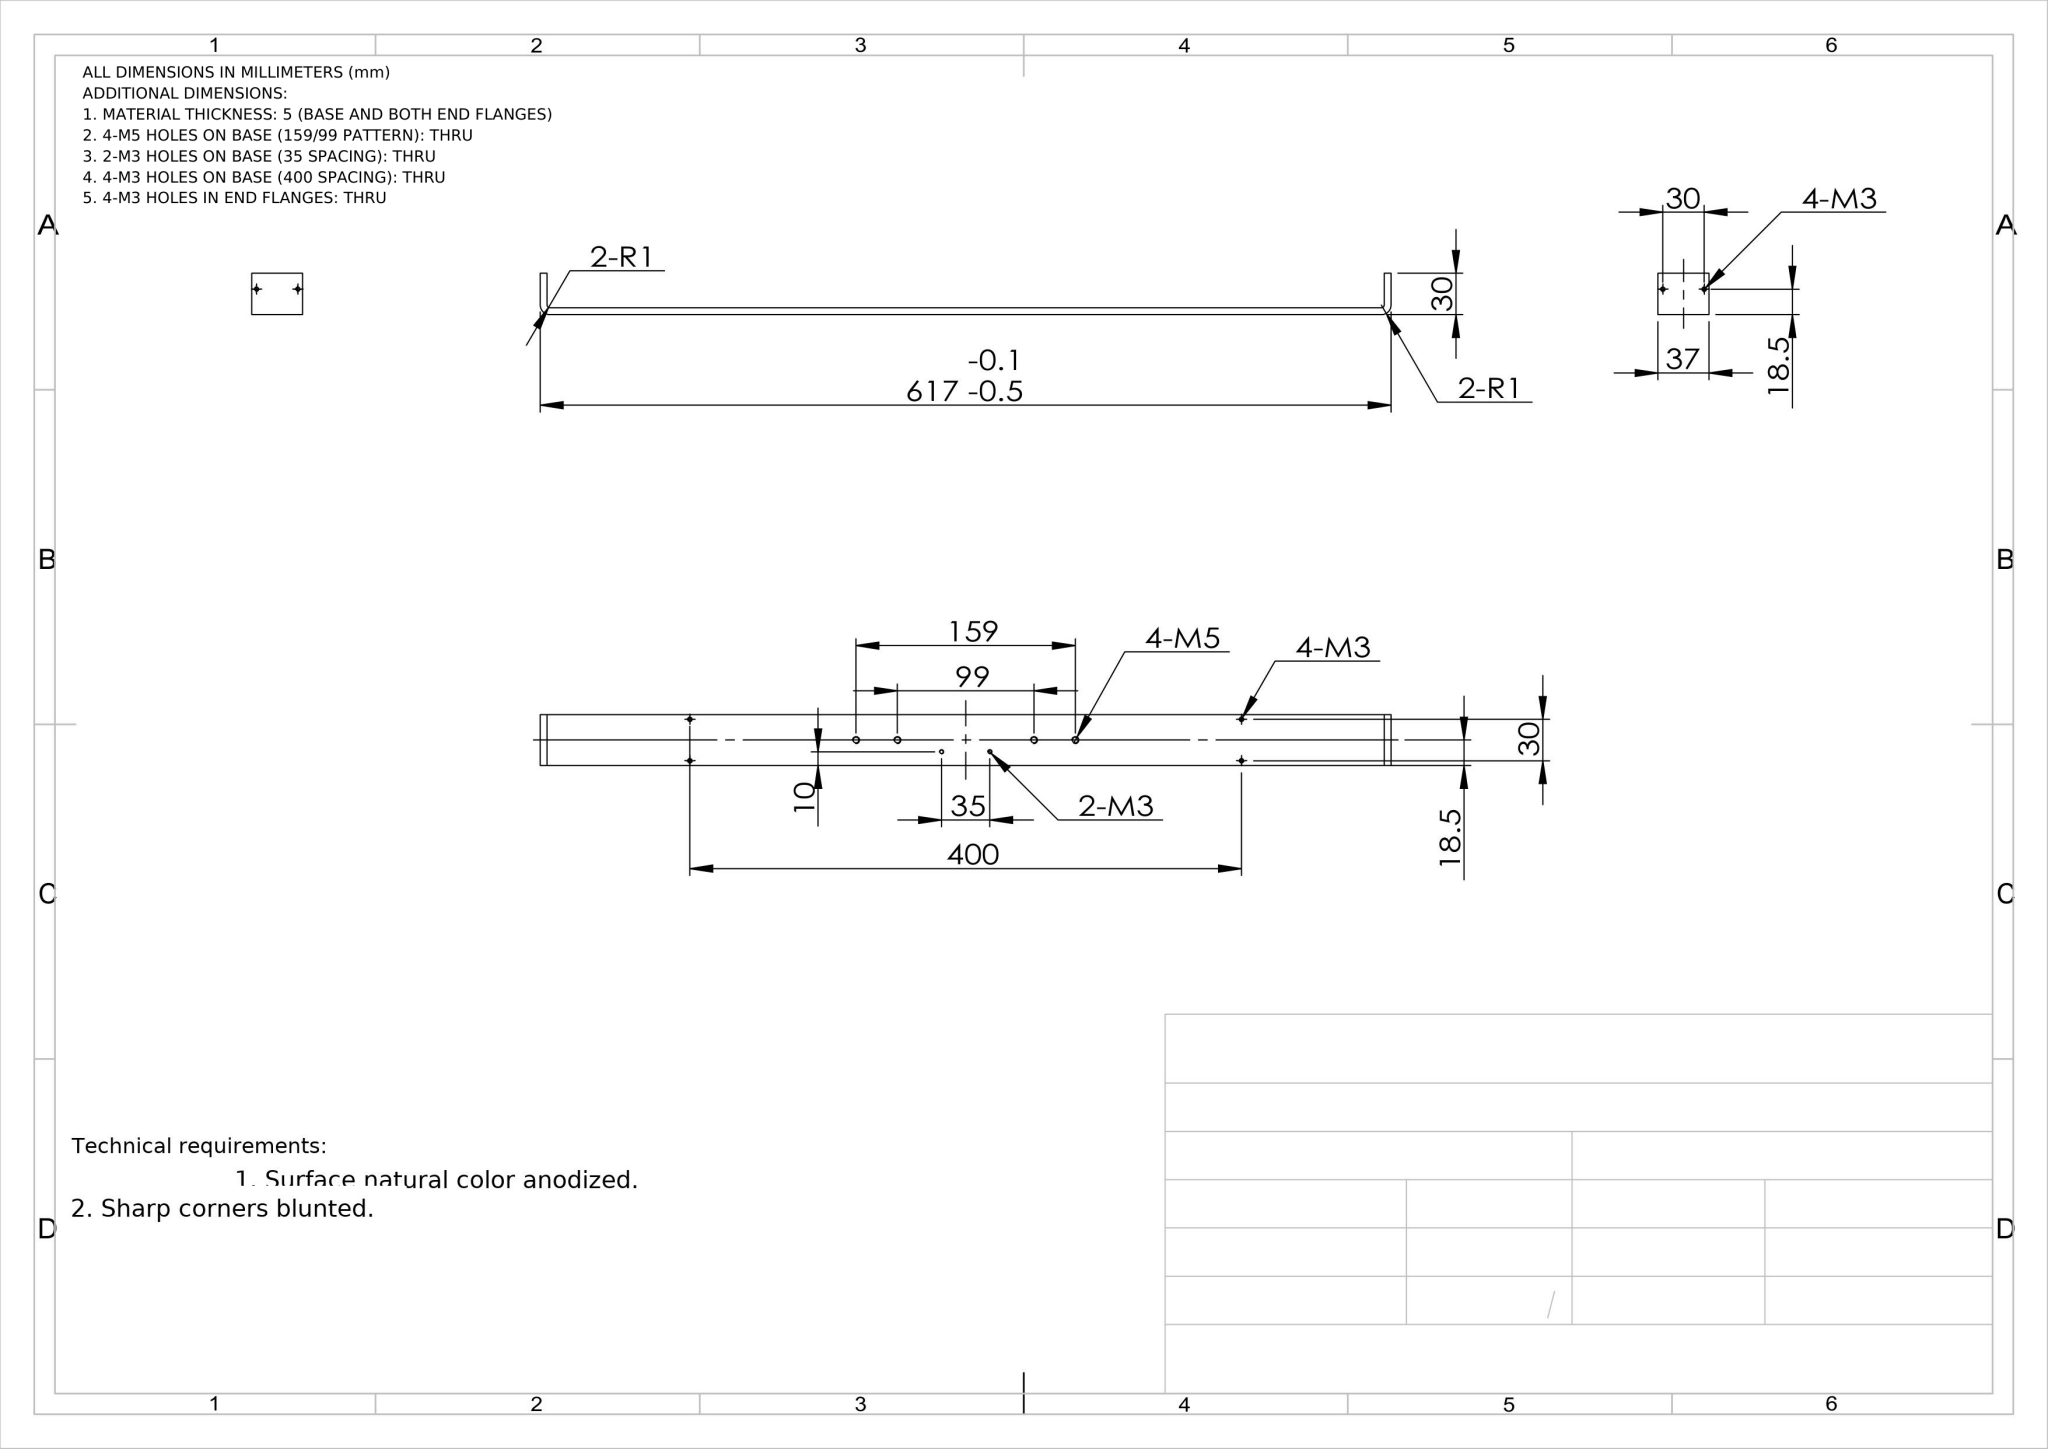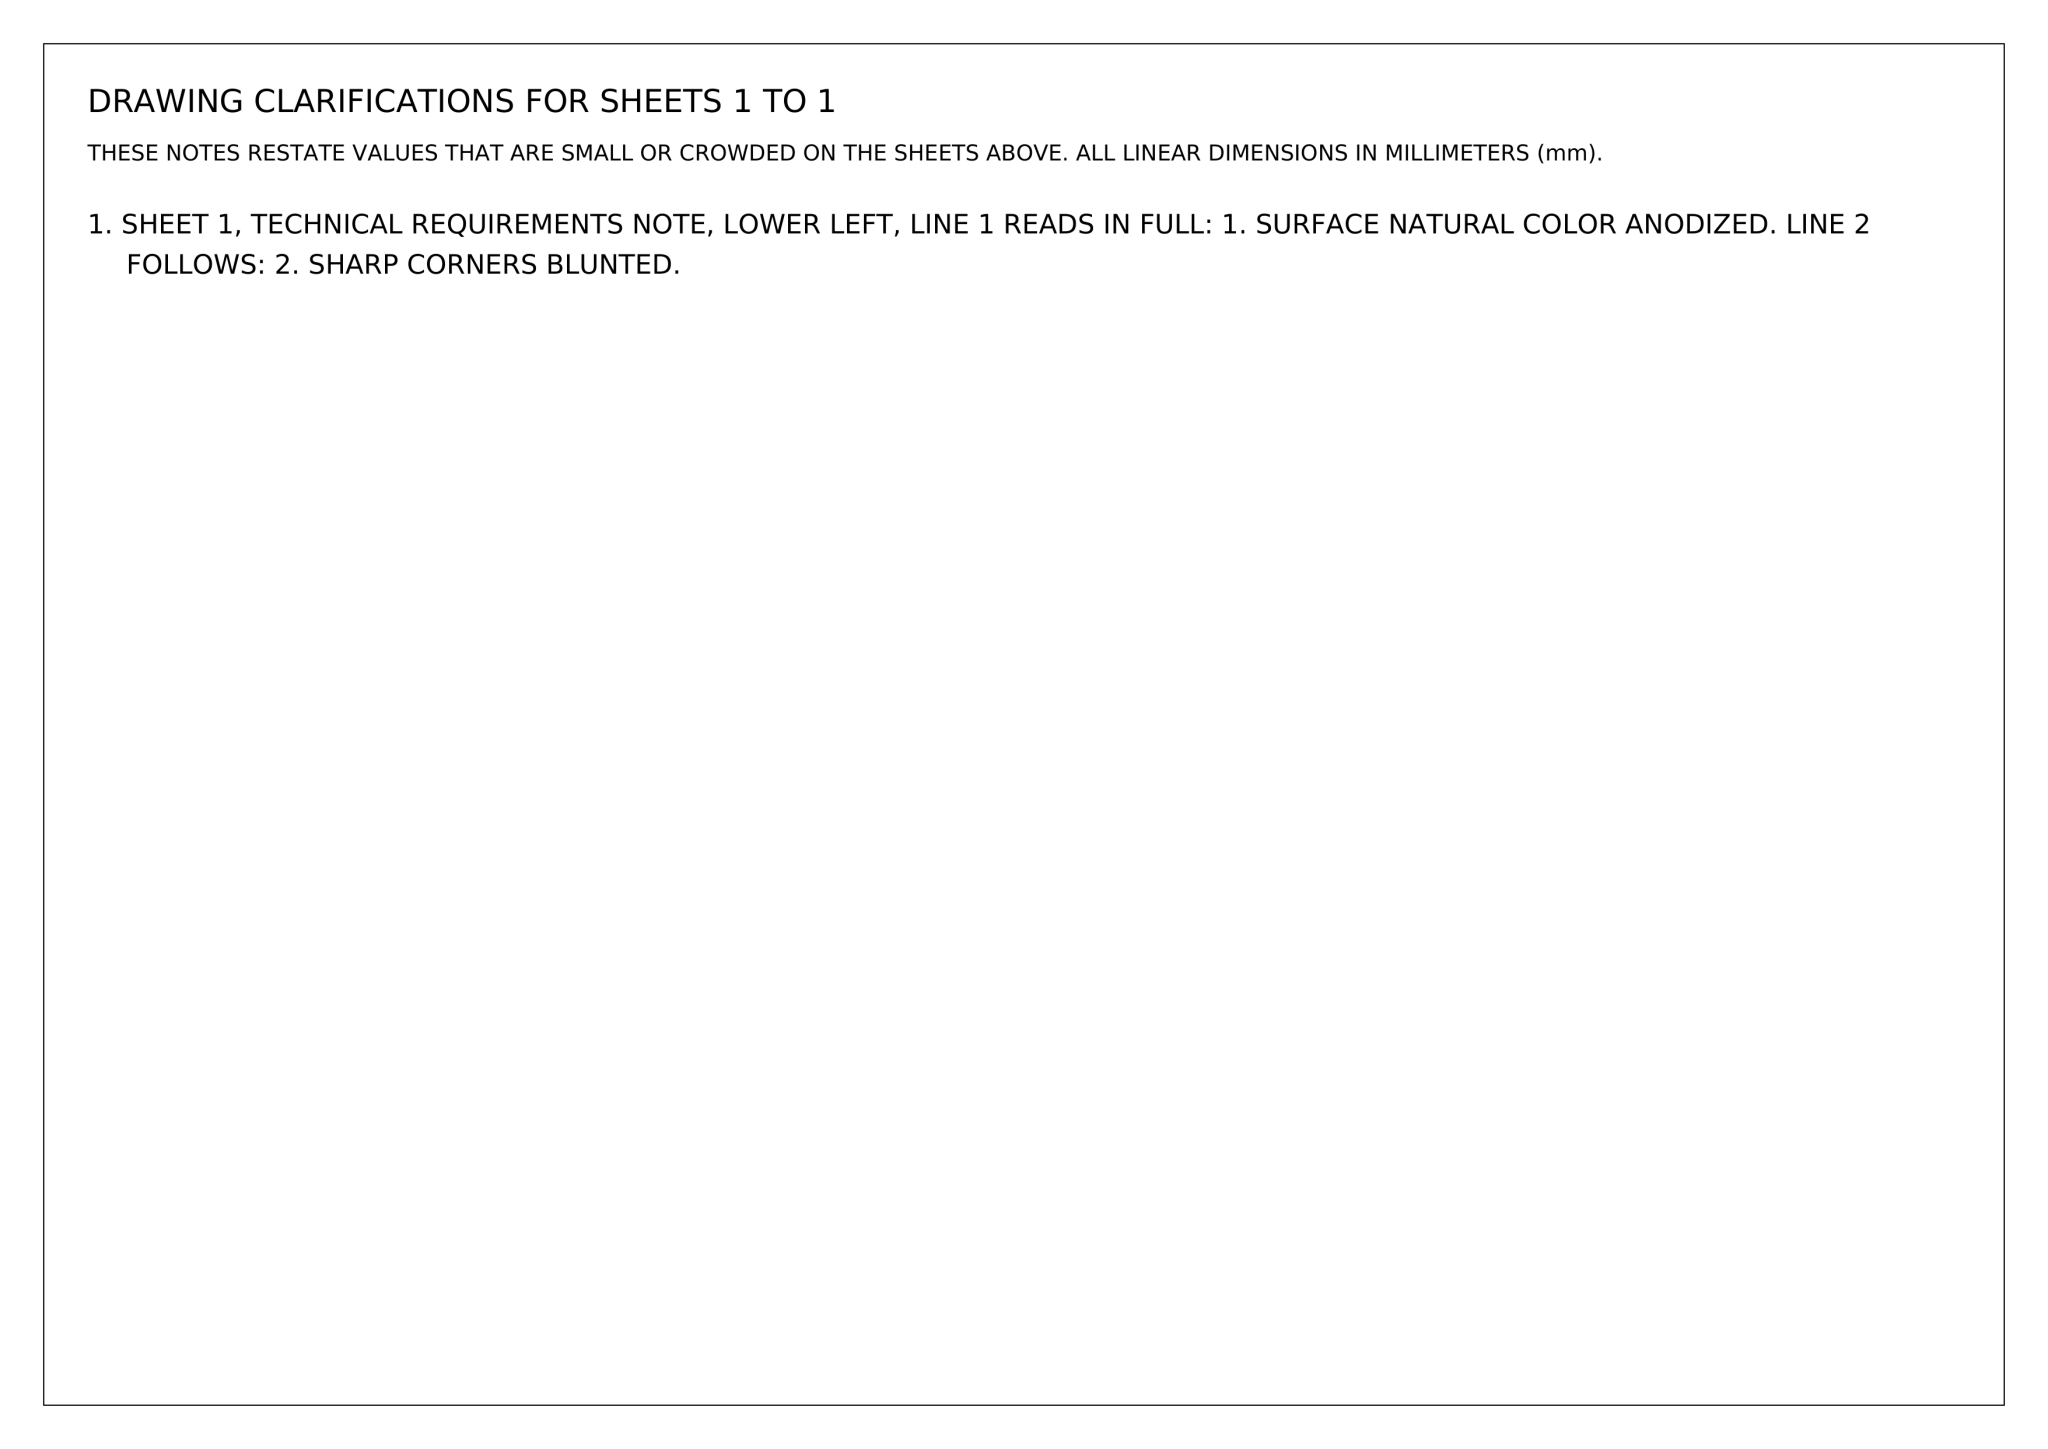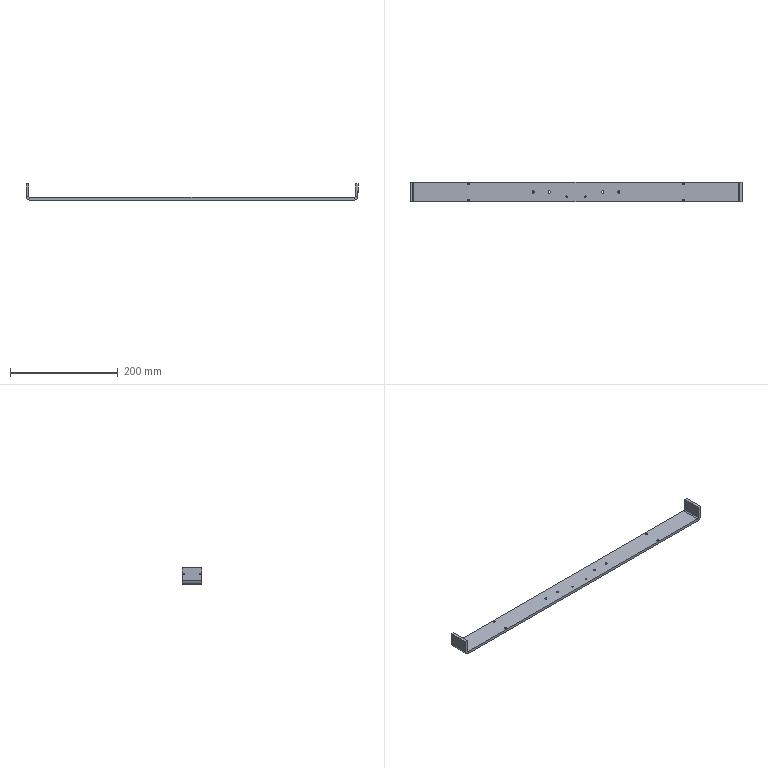Part | NX | mm | 1 solid | 70 faces | box 617 x 37 x 30 mm | volume 122151 mm3 | cylinder 32 | cone 20 | plane 18 | commonest cylinder face diameters 2.5 x20 4.2 x8 14 x2 4 x2